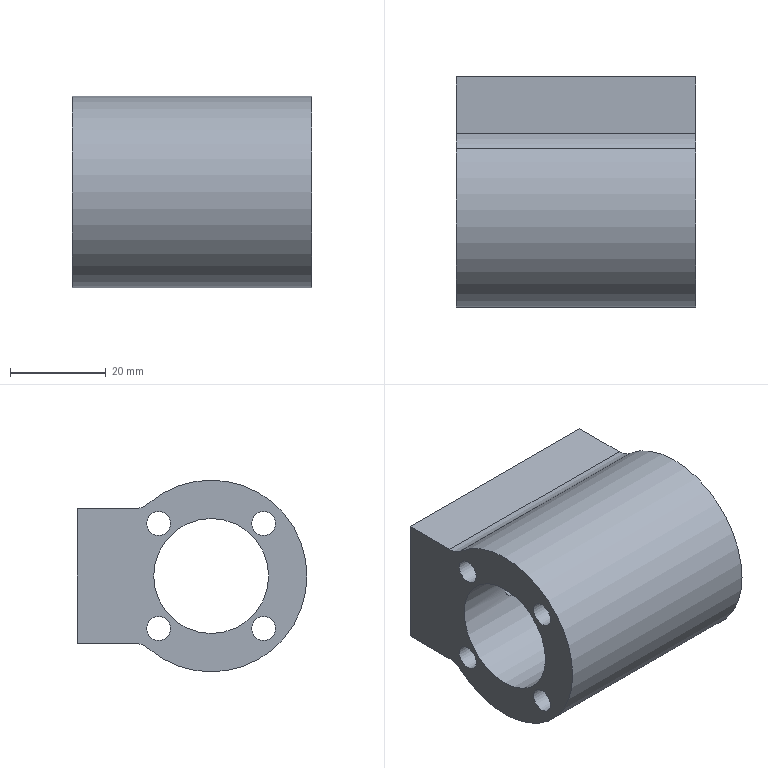Component | NX | EXTERNAL_PISTON_CYLINDER | 1 solid | 27 faces | volume 48967 mm3 | cylinder 14 | cone 8 | plane 5 | commonest cylinder face diameters 5 x6 4 x4 10 x2 24 x1 40 x1